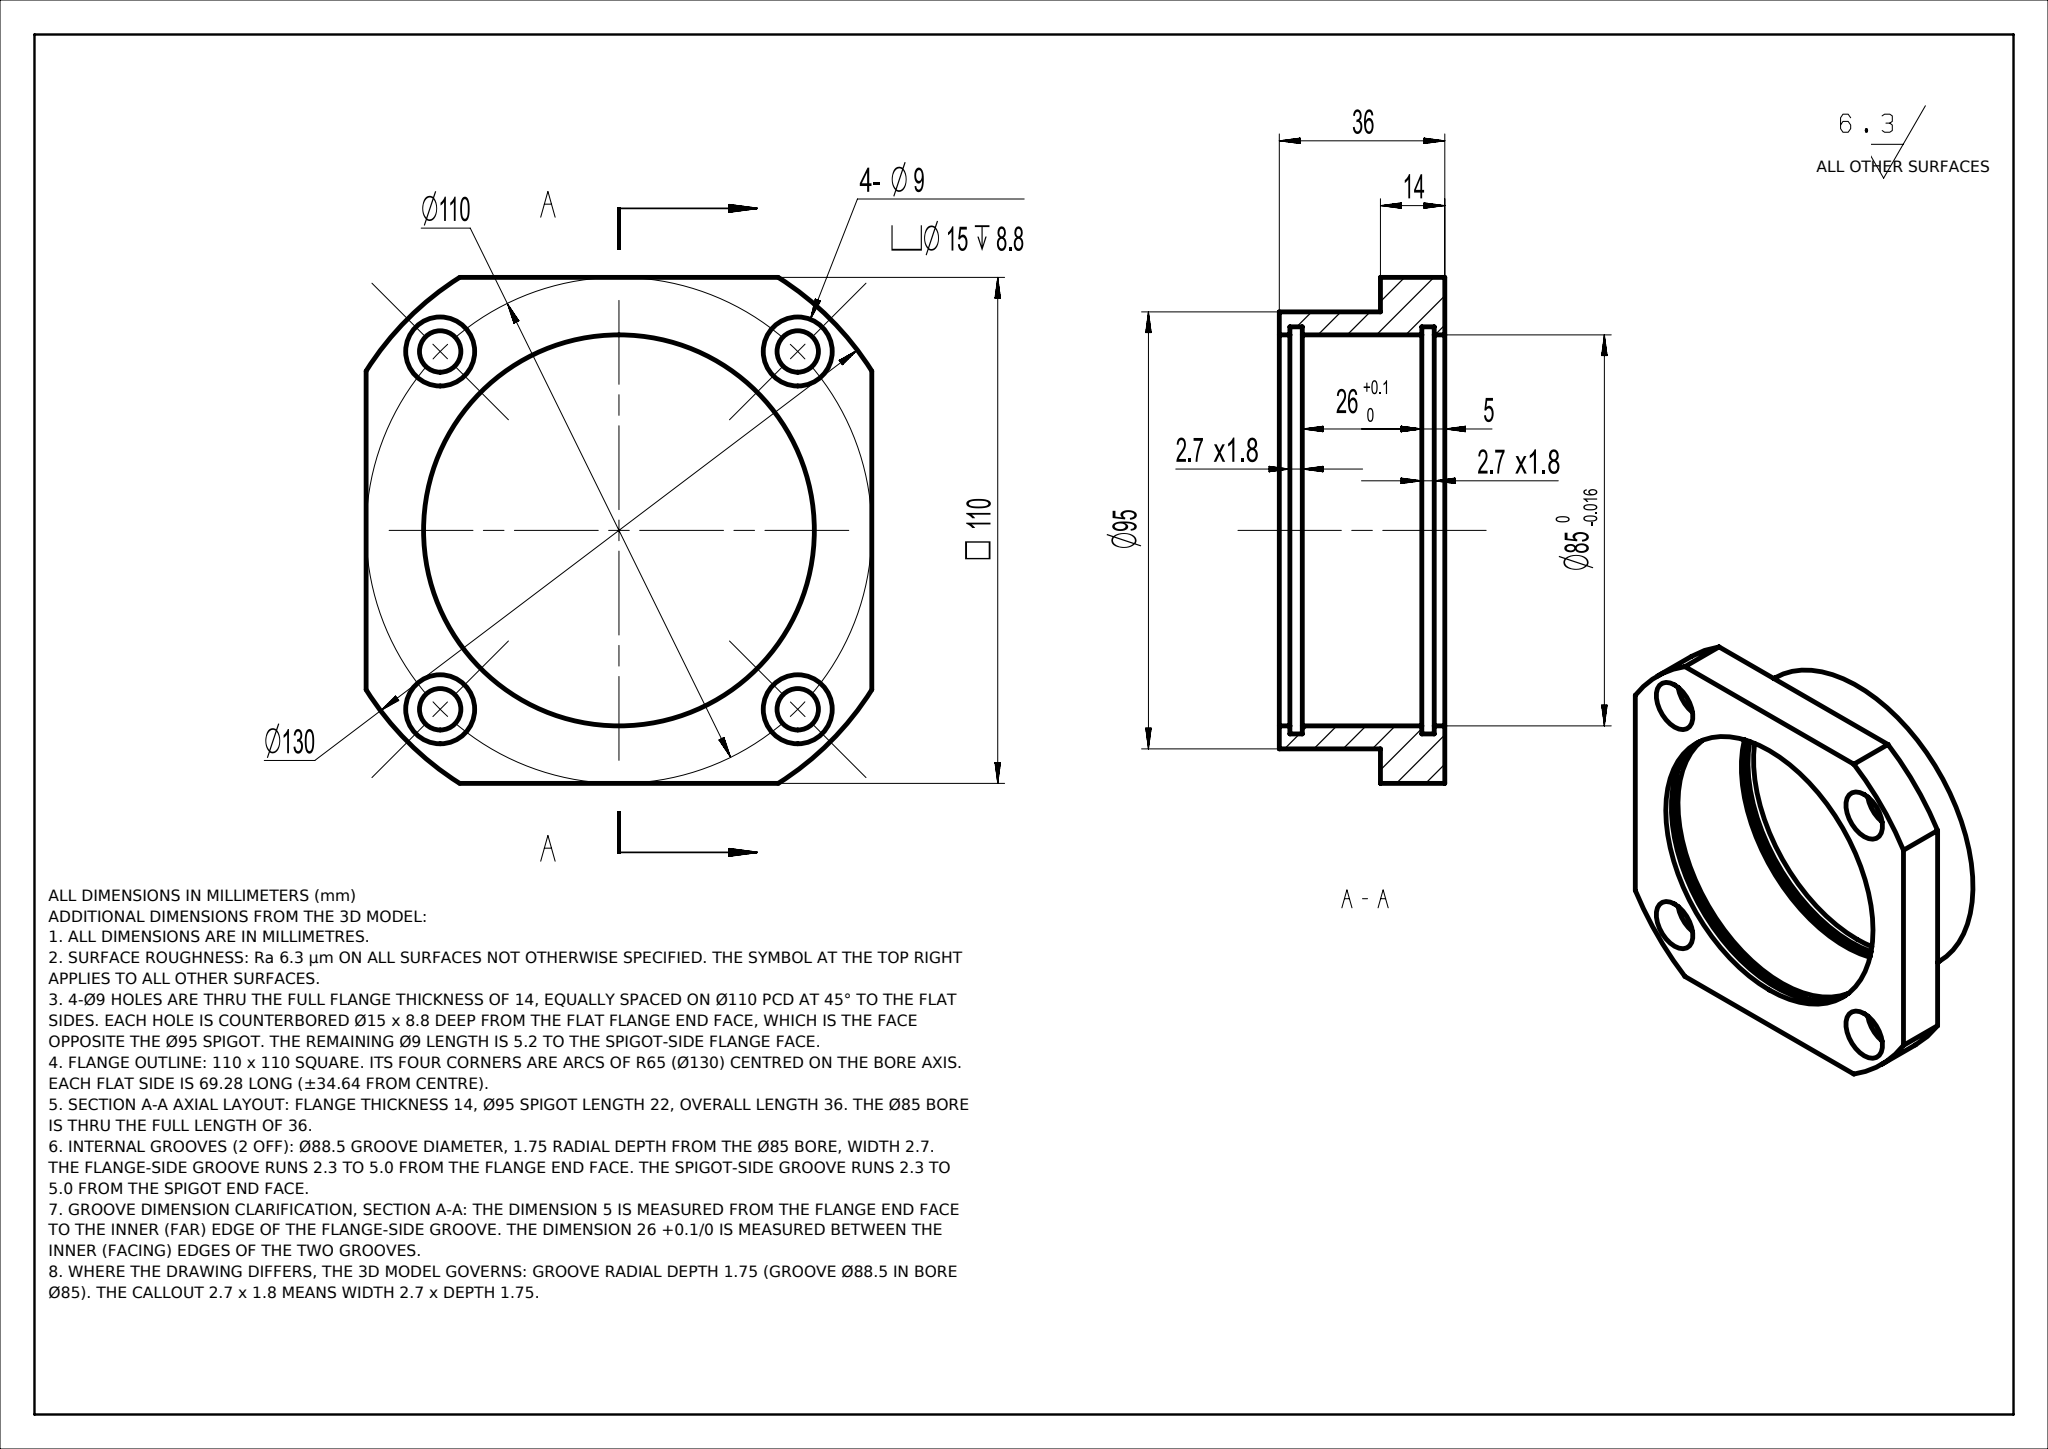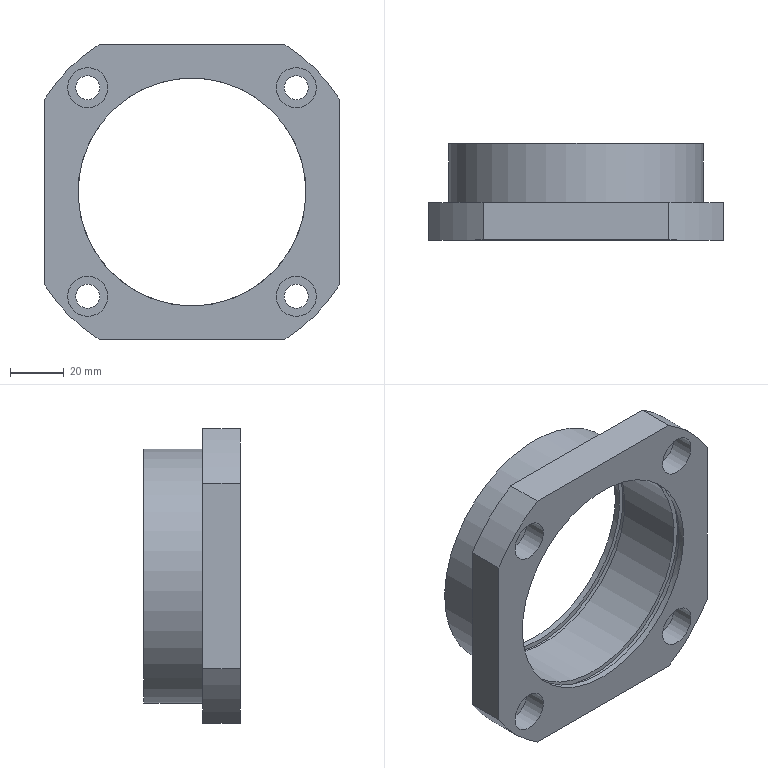Part | NX | mm | 1 solid | 33 faces | box 110 x 36 x 110 mm | volume 101074 mm3 | cylinder 18 | plane 15 | commonest cylinder face diameters 130 x4 9 x4 15 x4 85 x3 88.5 x2 95 x1
STEP:
#1=CARTESIAN_POINT('',(0.,0.,0.));
#2=DIRECTION('',(0.,0.,1.));
#3=DIRECTION('',(1.,0.,0.));
#4=AXIS2_PLACEMENT_3D('',#1,#2,#3);
#5=(LENGTH_UNIT()NAMED_UNIT(*)SI_UNIT(.MILLI.,.METRE.));
#6=UNCERTAINTY_MEASURE_WITH_UNIT(LENGTH_MEASURE(0.00002),#5,'','');
#7=(NAMED_UNIT(*)PLANE_ANGLE_UNIT()SI_UNIT($,.RADIAN.));
#8=PLANE_ANGLE_MEASURE_WITH_UNIT(PLANE_ANGLE_MEASURE(0.01745),#7);
#9=DIMENSIONAL_EXPONENTS(0.,0.,0.,0.,0.,0.,0.);
#10=(CONVERSION_BASED_UNIT('',#8)NAMED_UNIT(#9)PLANE_ANGLE_UNIT());
#11=(NAMED_UNIT(*)SI_UNIT($,.STERADIAN.)SOLID_ANGLE_UNIT());
#12=(GEOMETRIC_REPRESENTATION_CONTEXT(3)GLOBAL_UNCERTAINTY_ASSIGNED_CONTEXT((#6))GLOBAL_UNIT_ASSIGNED_CONTEXT((#5,#10,#11))REPRESENTATION_CONTEXT('',''));
#13=SHAPE_REPRESENTATION('',(#4),#12);
#14=CARTESIAN_POINT('',(-34.641,12.426,55.));
#15=VERTEX_POINT('',#14);
#16=CARTESIAN_POINT('',(-55.,12.426,34.641));
#17=VERTEX_POINT('',#16);
#18=CARTESIAN_POINT('',(0.,12.426,0.));
#19=DIRECTION('',(0.,-1.,0.));
#20=DIRECTION('',(0.,0.,-1.));
#21=AXIS2_PLACEMENT_3D('',#18,#19,#20);
#22=CIRCLE('',#21,65.);
#23=EDGE_CURVE('',#15,#17,#22,.T.);
#24=ORIENTED_EDGE('',*,*,#23,.T.);
#25=CARTESIAN_POINT('',(-55.,-1.574,34.641));
#26=VERTEX_POINT('',#25);
#27=CARTESIAN_POINT('',(-55.,0.,34.641));
#28=DIRECTION('',(0.,-1.,0.));
#29=VECTOR('',#28,1.);
#30=LINE('',#27,#29);
#31=EDGE_CURVE('',#17,#26,#30,.T.);
#32=ORIENTED_EDGE('',*,*,#31,.T.);
#33=CARTESIAN_POINT('',(-34.641,-1.574,55.));
#34=VERTEX_POINT('',#33);
#35=CARTESIAN_POINT('',(0.,-1.574,0.));
#36=DIRECTION('',(0.,-1.,0.));
#37=DIRECTION('',(0.,0.,-1.));
#38=AXIS2_PLACEMENT_3D('',#35,#36,#37);
#39=CIRCLE('',#38,65.);
#40=EDGE_CURVE('',#34,#26,#39,.T.);
#41=ORIENTED_EDGE('',*,*,#40,.F.);
#42=CARTESIAN_POINT('',(-34.641,0.,55.));
#43=DIRECTION('',(0.,1.,0.));
#44=VECTOR('',#43,1.);
#45=LINE('',#42,#44);
#46=EDGE_CURVE('',#34,#15,#45,.T.);
#47=ORIENTED_EDGE('',*,*,#46,.T.);
#48=EDGE_LOOP('',(#24,#32,#41,#47));
#49=FACE_OUTER_BOUND('',#48,.T.);
#50=CARTESIAN_POINT('',(0.,0.,0.));
#51=DIRECTION('',(0.,-1.,0.));
#52=DIRECTION('',(0.,0.,-1.));
#53=AXIS2_PLACEMENT_3D('',#50,#51,#52);
#54=CYLINDRICAL_SURFACE('',#53,65.);
#55=ADVANCED_FACE('',(#49),#54,.T.);
#56=CARTESIAN_POINT('',(-55.,-1.574,-34.641));
#57=VERTEX_POINT('',#56);
#58=CARTESIAN_POINT('',(-34.641,-1.574,-55.));
#59=VERTEX_POINT('',#58);
#60=CARTESIAN_POINT('',(0.,-1.574,0.));
#61=DIRECTION('',(0.,-1.,0.));
#62=DIRECTION('',(0.,0.,-1.));
#63=AXIS2_PLACEMENT_3D('',#60,#61,#62);
#64=CIRCLE('',#63,65.);
#65=EDGE_CURVE('',#57,#59,#64,.T.);
#66=ORIENTED_EDGE('',*,*,#65,.F.);
#67=CARTESIAN_POINT('',(-55.,12.426,-34.641));
#68=VERTEX_POINT('',#67);
#69=CARTESIAN_POINT('',(-55.,0.,-34.641));
#70=DIRECTION('',(0.,1.,0.));
#71=VECTOR('',#70,1.);
#72=LINE('',#69,#71);
#73=EDGE_CURVE('',#57,#68,#72,.T.);
#74=ORIENTED_EDGE('',*,*,#73,.T.);
#75=CARTESIAN_POINT('',(-34.641,12.426,-55.));
#76=VERTEX_POINT('',#75);
#77=CARTESIAN_POINT('',(0.,12.426,0.));
#78=DIRECTION('',(0.,-1.,0.));
#79=DIRECTION('',(0.,0.,-1.));
#80=AXIS2_PLACEMENT_3D('',#77,#78,#79);
#81=CIRCLE('',#80,65.);
#82=EDGE_CURVE('',#68,#76,#81,.T.);
#83=ORIENTED_EDGE('',*,*,#82,.T.);
#84=CARTESIAN_POINT('',(-34.641,0.,-55.));
#85=DIRECTION('',(0.,-1.,0.));
#86=VECTOR('',#85,1.);
#87=LINE('',#84,#86);
#88=EDGE_CURVE('',#76,#59,#87,.T.);
#89=ORIENTED_EDGE('',*,*,#88,.T.);
#90=EDGE_LOOP('',(#66,#74,#83,#89));
#91=FACE_OUTER_BOUND('',#90,.T.);
#92=CARTESIAN_POINT('',(0.,0.,0.));
#93=DIRECTION('',(0.,-1.,0.));
#94=DIRECTION('',(0.,0.,-1.));
#95=AXIS2_PLACEMENT_3D('',#92,#93,#94);
#96=CYLINDRICAL_SURFACE('',#95,65.);
#97=ADVANCED_FACE('',(#91),#96,.T.);
#98=CARTESIAN_POINT('',(34.641,-1.574,-55.));
#99=VERTEX_POINT('',#98);
#100=CARTESIAN_POINT('',(55.,-1.574,-34.641));
#101=VERTEX_POINT('',#100);
#102=CARTESIAN_POINT('',(0.,-1.574,0.));
#103=DIRECTION('',(0.,-1.,0.));
#104=DIRECTION('',(0.,0.,-1.));
#105=AXIS2_PLACEMENT_3D('',#102,#103,#104);
#106=CIRCLE('',#105,65.);
#107=EDGE_CURVE('',#99,#101,#106,.T.);
#108=ORIENTED_EDGE('',*,*,#107,.F.);
#109=CARTESIAN_POINT('',(34.641,12.426,-55.));
#110=VERTEX_POINT('',#109);
#111=CARTESIAN_POINT('',(34.641,0.,-55.));
#112=DIRECTION('',(0.,1.,0.));
#113=VECTOR('',#112,1.);
#114=LINE('',#111,#113);
#115=EDGE_CURVE('',#99,#110,#114,.T.);
#116=ORIENTED_EDGE('',*,*,#115,.T.);
#117=CARTESIAN_POINT('',(55.,12.426,-34.641));
#118=VERTEX_POINT('',#117);
#119=CARTESIAN_POINT('',(0.,12.426,0.));
#120=DIRECTION('',(0.,-1.,0.));
#121=DIRECTION('',(0.,0.,-1.));
#122=AXIS2_PLACEMENT_3D('',#119,#120,#121);
#123=CIRCLE('',#122,65.);
#124=EDGE_CURVE('',#110,#118,#123,.T.);
#125=ORIENTED_EDGE('',*,*,#124,.T.);
#126=CARTESIAN_POINT('',(55.,0.,-34.641));
#127=DIRECTION('',(0.,-1.,0.));
#128=VECTOR('',#127,1.);
#129=LINE('',#126,#128);
#130=EDGE_CURVE('',#118,#101,#129,.T.);
#131=ORIENTED_EDGE('',*,*,#130,.T.);
#132=EDGE_LOOP('',(#108,#116,#125,#131));
#133=FACE_OUTER_BOUND('',#132,.T.);
#134=CARTESIAN_POINT('',(0.,0.,0.));
#135=DIRECTION('',(0.,-1.,0.));
#136=DIRECTION('',(0.,0.,-1.));
#137=AXIS2_PLACEMENT_3D('',#134,#135,#136);
#138=CYLINDRICAL_SURFACE('',#137,65.);
#139=ADVANCED_FACE('',(#133),#138,.T.);
#140=CARTESIAN_POINT('',(0.,3.426,42.5));
#141=VERTEX_POINT('',#140);
#142=CARTESIAN_POINT('',(0.,3.426,0.));
#143=DIRECTION('',(0.,-1.,0.));
#144=DIRECTION('',(0.,0.,1.));
#145=AXIS2_PLACEMENT_3D('',#142,#143,#144);
#146=CIRCLE('',#145,42.5);
#147=EDGE_CURVE('',#141,#141,#146,.T.);
#148=ORIENTED_EDGE('',*,*,#147,.T.);
#149=EDGE_LOOP('',(#148));
#150=FACE_BOUND('',#149,.T.);
#151=CARTESIAN_POINT('',(0.,29.426,42.5));
#152=VERTEX_POINT('',#151);
#153=CARTESIAN_POINT('',(0.,29.426,0.));
#154=DIRECTION('',(0.,-1.,0.));
#155=DIRECTION('',(0.,0.,1.));
#156=AXIS2_PLACEMENT_3D('',#153,#154,#155);
#157=CIRCLE('',#156,42.5);
#158=EDGE_CURVE('',#152,#152,#157,.T.);
#159=ORIENTED_EDGE('',*,*,#158,.F.);
#160=EDGE_LOOP('',(#159));
#161=FACE_BOUND('',#160,.T.);
#162=CARTESIAN_POINT('',(0.,0.,0.));
#163=DIRECTION('',(0.,-1.,0.));
#164=DIRECTION('',(0.,0.,-1.));
#165=AXIS2_PLACEMENT_3D('',#162,#163,#164);
#166=CYLINDRICAL_SURFACE('',#165,42.5);
#167=ADVANCED_FACE('',(#150,#161),#166,.F.);
#168=CARTESIAN_POINT('',(0.,-1.574,-42.5));
#169=VERTEX_POINT('',#168);
#170=CARTESIAN_POINT('',(0.,-1.574,0.));
#171=DIRECTION('',(0.,-1.,0.));
#172=DIRECTION('',(0.,0.,-1.));
#173=AXIS2_PLACEMENT_3D('',#170,#171,#172);
#174=CIRCLE('',#173,42.5);
#175=EDGE_CURVE('',#169,#169,#174,.T.);
#176=ORIENTED_EDGE('',*,*,#175,.T.);
#177=EDGE_LOOP('',(#176));
#178=FACE_BOUND('',#177,.T.);
#179=CARTESIAN_POINT('',(0.,0.7259,42.5));
#180=VERTEX_POINT('',#179);
#181=CARTESIAN_POINT('',(0.,0.7259,0.));
#182=DIRECTION('',(0.,-1.,0.));
#183=DIRECTION('',(0.,0.,1.));
#184=AXIS2_PLACEMENT_3D('',#181,#182,#183);
#185=CIRCLE('',#184,42.5);
#186=EDGE_CURVE('',#180,#180,#185,.T.);
#187=ORIENTED_EDGE('',*,*,#186,.F.);
#188=EDGE_LOOP('',(#187));
#189=FACE_BOUND('',#188,.T.);
#190=CARTESIAN_POINT('',(0.,0.,0.));
#191=DIRECTION('',(0.,-1.,0.));
#192=DIRECTION('',(0.,0.,-1.));
#193=AXIS2_PLACEMENT_3D('',#190,#191,#192);
#194=CYLINDRICAL_SURFACE('',#193,42.5);
#195=ADVANCED_FACE('',(#178,#189),#194,.F.);
#196=CARTESIAN_POINT('',(38.891,-1.574,46.391));
#197=VERTEX_POINT('',#196);
#198=CARTESIAN_POINT('',(38.891,-1.574,38.891));
#199=DIRECTION('',(0.,1.,0.));
#200=DIRECTION('',(0.,0.,1.));
#201=AXIS2_PLACEMENT_3D('',#198,#199,#200);
#202=CIRCLE('',#201,7.5);
#203=EDGE_CURVE('',#197,#197,#202,.T.);
#204=ORIENTED_EDGE('',*,*,#203,.T.);
#205=EDGE_LOOP('',(#204));
#206=FACE_BOUND('',#205,.T.);
#207=CARTESIAN_POINT('',(38.891,-1.574,-31.391));
#208=VERTEX_POINT('',#207);
#209=CARTESIAN_POINT('',(38.891,-1.574,-38.891));
#210=DIRECTION('',(0.,1.,0.));
#211=DIRECTION('',(0.,0.,1.));
#212=AXIS2_PLACEMENT_3D('',#209,#210,#211);
#213=CIRCLE('',#212,7.5);
#214=EDGE_CURVE('',#208,#208,#213,.T.);
#215=ORIENTED_EDGE('',*,*,#214,.T.);
#216=EDGE_LOOP('',(#215));
#217=FACE_BOUND('',#216,.T.);
#218=CARTESIAN_POINT('',(-38.891,-1.574,46.391));
#219=VERTEX_POINT('',#218);
#220=CARTESIAN_POINT('',(-38.891,-1.574,38.891));
#221=DIRECTION('',(0.,1.,0.));
#222=DIRECTION('',(0.,0.,1.));
#223=AXIS2_PLACEMENT_3D('',#220,#221,#222);
#224=CIRCLE('',#223,7.5);
#225=EDGE_CURVE('',#219,#219,#224,.T.);
#226=ORIENTED_EDGE('',*,*,#225,.T.);
#227=EDGE_LOOP('',(#226));
#228=FACE_BOUND('',#227,.T.);
#229=CARTESIAN_POINT('',(-38.891,-1.574,-31.391));
#230=VERTEX_POINT('',#229);
#231=CARTESIAN_POINT('',(-38.891,-1.574,-38.891));
#232=DIRECTION('',(0.,1.,0.));
#233=DIRECTION('',(0.,0.,1.));
#234=AXIS2_PLACEMENT_3D('',#231,#232,#233);
#235=CIRCLE('',#234,7.5);
#236=EDGE_CURVE('',#230,#230,#235,.T.);
#237=ORIENTED_EDGE('',*,*,#236,.T.);
#238=EDGE_LOOP('',(#237));
#239=FACE_BOUND('',#238,.T.);
#240=ORIENTED_EDGE('',*,*,#175,.F.);
#241=EDGE_LOOP('',(#240));
#242=FACE_BOUND('',#241,.T.);
#243=CARTESIAN_POINT('',(55.,-1.574,34.641));
#244=VERTEX_POINT('',#243);
#245=CARTESIAN_POINT('',(34.641,-1.574,55.));
#246=VERTEX_POINT('',#245);
#247=CARTESIAN_POINT('',(0.,-1.574,0.));
#248=DIRECTION('',(0.,-1.,0.));
#249=DIRECTION('',(0.,0.,-1.));
#250=AXIS2_PLACEMENT_3D('',#247,#248,#249);
#251=CIRCLE('',#250,65.);
#252=EDGE_CURVE('',#244,#246,#251,.T.);
#253=ORIENTED_EDGE('',*,*,#252,.T.);
#254=CARTESIAN_POINT('',(55.,-1.574,55.));
#255=DIRECTION('',(-1.,0.,0.));
#256=VECTOR('',#255,1.);
#257=LINE('',#254,#256);
#258=EDGE_CURVE('',#246,#34,#257,.T.);
#259=ORIENTED_EDGE('',*,*,#258,.T.);
#260=ORIENTED_EDGE('',*,*,#40,.T.);
#261=CARTESIAN_POINT('',(-55.,-1.574,55.));
#262=DIRECTION('',(-0.,0.,-1.));
#263=VECTOR('',#262,1.);
#264=LINE('',#261,#263);
#265=EDGE_CURVE('',#26,#57,#264,.T.);
#266=ORIENTED_EDGE('',*,*,#265,.T.);
#267=ORIENTED_EDGE('',*,*,#65,.T.);
#268=CARTESIAN_POINT('',(-55.,-1.574,-55.));
#269=DIRECTION('',(1.,0.,-0.));
#270=VECTOR('',#269,1.);
#271=LINE('',#268,#270);
#272=EDGE_CURVE('',#59,#99,#271,.T.);
#273=ORIENTED_EDGE('',*,*,#272,.T.);
#274=ORIENTED_EDGE('',*,*,#107,.T.);
#275=CARTESIAN_POINT('',(55.,-1.574,-55.));
#276=DIRECTION('',(0.,0.,1.));
#277=VECTOR('',#276,1.);
#278=LINE('',#275,#277);
#279=EDGE_CURVE('',#101,#244,#278,.T.);
#280=ORIENTED_EDGE('',*,*,#279,.T.);
#281=EDGE_LOOP('',(#253,#259,#260,#266,#267,#273,#274,#280));
#282=FACE_BOUND('',#281,.T.);
#283=CARTESIAN_POINT('',(0.,-1.574,65.));
#284=DIRECTION('',(0.,1.,0.));
#285=DIRECTION('',(0.,0.,1.));
#286=AXIS2_PLACEMENT_3D('',#283,#284,#285);
#287=PLANE('',#286);
#288=ADVANCED_FACE('',(#206,#217,#228,#239,#242,#282),#287,.F.);
#289=CARTESIAN_POINT('',(0.,32.126,42.5));
#290=VERTEX_POINT('',#289);
#291=CARTESIAN_POINT('',(0.,32.126,0.));
#292=DIRECTION('',(0.,-1.,0.));
#293=DIRECTION('',(0.,0.,1.));
#294=AXIS2_PLACEMENT_3D('',#291,#292,#293);
#295=CIRCLE('',#294,42.5);
#296=EDGE_CURVE('',#290,#290,#295,.T.);
#297=ORIENTED_EDGE('',*,*,#296,.T.);
#298=EDGE_LOOP('',(#297));
#299=FACE_BOUND('',#298,.T.);
#300=CARTESIAN_POINT('',(0.,34.426,-42.5));
#301=VERTEX_POINT('',#300);
#302=CARTESIAN_POINT('',(0.,34.426,0.));
#303=DIRECTION('',(0.,-1.,0.));
#304=DIRECTION('',(0.,0.,-1.));
#305=AXIS2_PLACEMENT_3D('',#302,#303,#304);
#306=CIRCLE('',#305,42.5);
#307=EDGE_CURVE('',#301,#301,#306,.T.);
#308=ORIENTED_EDGE('',*,*,#307,.F.);
#309=EDGE_LOOP('',(#308));
#310=FACE_BOUND('',#309,.T.);
#311=CARTESIAN_POINT('',(0.,0.,0.));
#312=DIRECTION('',(0.,-1.,0.));
#313=DIRECTION('',(0.,0.,-1.));
#314=AXIS2_PLACEMENT_3D('',#311,#312,#313);
#315=CYLINDRICAL_SURFACE('',#314,42.5);
#316=ADVANCED_FACE('',(#299,#310),#315,.F.);
#317=CARTESIAN_POINT('',(0.,34.426,-47.5));
#318=VERTEX_POINT('',#317);
#319=CARTESIAN_POINT('',(0.,34.426,0.));
#320=DIRECTION('',(0.,-1.,0.));
#321=DIRECTION('',(0.,0.,-1.));
#322=AXIS2_PLACEMENT_3D('',#319,#320,#321);
#323=CIRCLE('',#322,47.5);
#324=EDGE_CURVE('',#318,#318,#323,.T.);
#325=ORIENTED_EDGE('',*,*,#324,.F.);
#326=EDGE_LOOP('',(#325));
#327=FACE_BOUND('',#326,.T.);
#328=ORIENTED_EDGE('',*,*,#307,.T.);
#329=EDGE_LOOP('',(#328));
#330=FACE_BOUND('',#329,.T.);
#331=CARTESIAN_POINT('',(0.,34.426,42.5));
#332=DIRECTION('',(0.,-1.,0.));
#333=DIRECTION('',(0.,0.,-1.));
#334=AXIS2_PLACEMENT_3D('',#331,#332,#333);
#335=PLANE('',#334);
#336=ADVANCED_FACE('',(#327,#330),#335,.F.);
#337=CARTESIAN_POINT('',(0.,12.426,-47.5));
#338=VERTEX_POINT('',#337);
#339=CARTESIAN_POINT('',(0.,12.426,0.));
#340=DIRECTION('',(0.,-1.,0.));
#341=DIRECTION('',(0.,0.,-1.));
#342=AXIS2_PLACEMENT_3D('',#339,#340,#341);
#343=CIRCLE('',#342,47.5);
#344=EDGE_CURVE('',#338,#338,#343,.T.);
#345=ORIENTED_EDGE('',*,*,#344,.F.);
#346=EDGE_LOOP('',(#345));
#347=FACE_BOUND('',#346,.T.);
#348=ORIENTED_EDGE('',*,*,#324,.T.);
#349=EDGE_LOOP('',(#348));
#350=FACE_BOUND('',#349,.T.);
#351=CARTESIAN_POINT('',(0.,0.,0.));
#352=DIRECTION('',(0.,-1.,0.));
#353=DIRECTION('',(0.,0.,-1.));
#354=AXIS2_PLACEMENT_3D('',#351,#352,#353);
#355=CYLINDRICAL_SURFACE('',#354,47.5);
#356=ADVANCED_FACE('',(#347,#350),#355,.T.);
#357=CARTESIAN_POINT('',(38.891,12.426,34.391));
#358=VERTEX_POINT('',#357);
#359=CARTESIAN_POINT('',(38.891,12.426,38.891));
#360=DIRECTION('',(0.,-1.,0.));
#361=DIRECTION('',(0.,0.,-1.));
#362=AXIS2_PLACEMENT_3D('',#359,#360,#361);
#363=CIRCLE('',#362,4.5);
#364=EDGE_CURVE('',#358,#358,#363,.T.);
#365=ORIENTED_EDGE('',*,*,#364,.T.);
#366=EDGE_LOOP('',(#365));
#367=FACE_BOUND('',#366,.T.);
#368=CARTESIAN_POINT('',(38.891,12.426,-43.391));
#369=VERTEX_POINT('',#368);
#370=CARTESIAN_POINT('',(38.891,12.426,-38.891));
#371=DIRECTION('',(0.,-1.,0.));
#372=DIRECTION('',(0.,0.,-1.));
#373=AXIS2_PLACEMENT_3D('',#370,#371,#372);
#374=CIRCLE('',#373,4.5);
#375=EDGE_CURVE('',#369,#369,#374,.T.);
#376=ORIENTED_EDGE('',*,*,#375,.T.);
#377=EDGE_LOOP('',(#376));
#378=FACE_BOUND('',#377,.T.);
#379=CARTESIAN_POINT('',(-38.891,12.426,34.391));
#380=VERTEX_POINT('',#379);
#381=CARTESIAN_POINT('',(-38.891,12.426,38.891));
#382=DIRECTION('',(0.,-1.,0.));
#383=DIRECTION('',(0.,0.,-1.));
#384=AXIS2_PLACEMENT_3D('',#381,#382,#383);
#385=CIRCLE('',#384,4.5);
#386=EDGE_CURVE('',#380,#380,#385,.T.);
#387=ORIENTED_EDGE('',*,*,#386,.T.);
#388=EDGE_LOOP('',(#387));
#389=FACE_BOUND('',#388,.T.);
#390=CARTESIAN_POINT('',(-38.891,12.426,-43.391));
#391=VERTEX_POINT('',#390);
#392=CARTESIAN_POINT('',(-38.891,12.426,-38.891));
#393=DIRECTION('',(0.,-1.,0.));
#394=DIRECTION('',(0.,0.,-1.));
#395=AXIS2_PLACEMENT_3D('',#392,#393,#394);
#396=CIRCLE('',#395,4.5);
#397=EDGE_CURVE('',#391,#391,#396,.T.);
#398=ORIENTED_EDGE('',*,*,#397,.T.);
#399=EDGE_LOOP('',(#398));
#400=FACE_BOUND('',#399,.T.);
#401=ORIENTED_EDGE('',*,*,#82,.F.);
#402=CARTESIAN_POINT('',(-55.,12.426,47.5));
#403=DIRECTION('',(0.,0.,1.));
#404=VECTOR('',#403,1.);
#405=LINE('',#402,#404);
#406=EDGE_CURVE('',#68,#17,#405,.T.);
#407=ORIENTED_EDGE('',*,*,#406,.T.);
#408=ORIENTED_EDGE('',*,*,#23,.F.);
#409=CARTESIAN_POINT('',(34.641,12.426,55.));
#410=VERTEX_POINT('',#409);
#411=CARTESIAN_POINT('',(0.,12.426,55.));
#412=DIRECTION('',(1.,0.,-0.));
#413=VECTOR('',#412,1.);
#414=LINE('',#411,#413);
#415=EDGE_CURVE('',#15,#410,#414,.T.);
#416=ORIENTED_EDGE('',*,*,#415,.T.);
#417=CARTESIAN_POINT('',(55.,12.426,34.641));
#418=VERTEX_POINT('',#417);
#419=CARTESIAN_POINT('',(0.,12.426,0.));
#420=DIRECTION('',(0.,-1.,0.));
#421=DIRECTION('',(0.,0.,-1.));
#422=AXIS2_PLACEMENT_3D('',#419,#420,#421);
#423=CIRCLE('',#422,65.);
#424=EDGE_CURVE('',#418,#410,#423,.T.);
#425=ORIENTED_EDGE('',*,*,#424,.F.);
#426=CARTESIAN_POINT('',(55.,12.426,47.5));
#427=DIRECTION('',(-0.,0.,-1.));
#428=VECTOR('',#427,1.);
#429=LINE('',#426,#428);
#430=EDGE_CURVE('',#418,#118,#429,.T.);
#431=ORIENTED_EDGE('',*,*,#430,.T.);
#432=ORIENTED_EDGE('',*,*,#124,.F.);
#433=CARTESIAN_POINT('',(-0.,12.426,-55.));
#434=DIRECTION('',(-1.,0.,0.));
#435=VECTOR('',#434,1.);
#436=LINE('',#433,#435);
#437=EDGE_CURVE('',#110,#76,#436,.T.);
#438=ORIENTED_EDGE('',*,*,#437,.T.);
#439=EDGE_LOOP('',(#401,#407,#408,#416,#425,#431,#432,#438));
#440=FACE_BOUND('',#439,.T.);
#441=ORIENTED_EDGE('',*,*,#344,.T.);
#442=EDGE_LOOP('',(#441));
#443=FACE_BOUND('',#442,.T.);
#444=CARTESIAN_POINT('',(0.,12.426,47.5));
#445=DIRECTION('',(0.,-1.,0.));
#446=DIRECTION('',(0.,0.,-1.));
#447=AXIS2_PLACEMENT_3D('',#444,#445,#446);
#448=PLANE('',#447);
#449=ADVANCED_FACE('',(#367,#378,#389,#400,#440,#443),#448,.F.);
#450=ORIENTED_EDGE('',*,*,#252,.F.);
#451=CARTESIAN_POINT('',(55.,0.,34.641));
#452=DIRECTION('',(0.,1.,0.));
#453=VECTOR('',#452,1.);
#454=LINE('',#451,#453);
#455=EDGE_CURVE('',#244,#418,#454,.T.);
#456=ORIENTED_EDGE('',*,*,#455,.T.);
#457=ORIENTED_EDGE('',*,*,#424,.T.);
#458=CARTESIAN_POINT('',(34.641,0.,55.));
#459=DIRECTION('',(0.,-1.,0.));
#460=VECTOR('',#459,1.);
#461=LINE('',#458,#460);
#462=EDGE_CURVE('',#410,#246,#461,.T.);
#463=ORIENTED_EDGE('',*,*,#462,.T.);
#464=EDGE_LOOP('',(#450,#456,#457,#463));
#465=FACE_OUTER_BOUND('',#464,.T.);
#466=CARTESIAN_POINT('',(0.,0.,0.));
#467=DIRECTION('',(0.,-1.,0.));
#468=DIRECTION('',(0.,0.,-1.));
#469=AXIS2_PLACEMENT_3D('',#466,#467,#468);
#470=CYLINDRICAL_SURFACE('',#469,65.);
#471=ADVANCED_FACE('',(#465),#470,.T.);
#472=CARTESIAN_POINT('',(0.,0.7259,44.25));
#473=VERTEX_POINT('',#472);
#474=CARTESIAN_POINT('',(0.,0.7259,0.));
#475=DIRECTION('',(0.,-1.,0.));
#476=DIRECTION('',(0.,0.,1.));
#477=AXIS2_PLACEMENT_3D('',#474,#475,#476);
#478=CIRCLE('',#477,44.25);
#479=EDGE_CURVE('',#473,#473,#478,.T.);
#480=ORIENTED_EDGE('',*,*,#479,.F.);
#481=EDGE_LOOP('',(#480));
#482=FACE_BOUND('',#481,.T.);
#483=ORIENTED_EDGE('',*,*,#186,.T.);
#484=EDGE_LOOP('',(#483));
#485=FACE_BOUND('',#484,.T.);
#486=CARTESIAN_POINT('',(0.,0.7259,0.));
#487=DIRECTION('',(0.,1.,0.));
#488=DIRECTION('',(0.,0.,1.));
#489=AXIS2_PLACEMENT_3D('',#486,#487,#488);
#490=PLANE('',#489);
#491=ADVANCED_FACE('',(#482,#485),#490,.T.);
#492=CARTESIAN_POINT('',(0.,3.426,44.25));
#493=VERTEX_POINT('',#492);
#494=CARTESIAN_POINT('',(0.,3.426,0.));
#495=DIRECTION('',(0.,-1.,0.));
#496=DIRECTION('',(0.,0.,1.));
#497=AXIS2_PLACEMENT_3D('',#494,#495,#496);
#498=CIRCLE('',#497,44.25);
#499=EDGE_CURVE('',#493,#493,#498,.T.);
#500=ORIENTED_EDGE('',*,*,#499,.T.);
#501=EDGE_LOOP('',(#500));
#502=FACE_BOUND('',#501,.T.);
#503=ORIENTED_EDGE('',*,*,#147,.F.);
#504=EDGE_LOOP('',(#503));
#505=FACE_BOUND('',#504,.T.);
#506=CARTESIAN_POINT('',(0.,3.426,0.));
#507=DIRECTION('',(0.,1.,0.));
#508=DIRECTION('',(0.,0.,1.));
#509=AXIS2_PLACEMENT_3D('',#506,#507,#508);
#510=PLANE('',#509);
#511=ADVANCED_FACE('',(#502,#505),#510,.F.);
#512=ORIENTED_EDGE('',*,*,#499,.F.);
#513=EDGE_LOOP('',(#512));
#514=FACE_BOUND('',#513,.T.);
#515=ORIENTED_EDGE('',*,*,#479,.T.);
#516=EDGE_LOOP('',(#515));
#517=FACE_BOUND('',#516,.T.);
#518=CARTESIAN_POINT('',(0.,2.076,0.));
#519=DIRECTION('',(0.,1.,0.));
#520=DIRECTION('',(0.,0.,1.));
#521=AXIS2_PLACEMENT_3D('',#518,#519,#520);
#522=CYLINDRICAL_SURFACE('',#521,44.25);
#523=ADVANCED_FACE('',(#514,#517),#522,.F.);
#524=CARTESIAN_POINT('',(0.,32.126,44.25));
#525=VERTEX_POINT('',#524);
#526=CARTESIAN_POINT('',(0.,32.126,0.));
#527=DIRECTION('',(0.,-1.,0.));
#528=DIRECTION('',(0.,0.,1.));
#529=AXIS2_PLACEMENT_3D('',#526,#527,#528);
#530=CIRCLE('',#529,44.25);
#531=EDGE_CURVE('',#525,#525,#530,.T.);
#532=ORIENTED_EDGE('',*,*,#531,.T.);
#533=EDGE_LOOP('',(#532));
#534=FACE_BOUND('',#533,.T.);
#535=ORIENTED_EDGE('',*,*,#296,.F.);
#536=EDGE_LOOP('',(#535));
#537=FACE_BOUND('',#536,.T.);
#538=CARTESIAN_POINT('',(0.,32.126,0.));
#539=DIRECTION('',(0.,1.,0.));
#540=DIRECTION('',(0.,0.,1.));
#541=AXIS2_PLACEMENT_3D('',#538,#539,#540);
#542=PLANE('',#541);
#543=ADVANCED_FACE('',(#534,#537),#542,.F.);
#544=CARTESIAN_POINT('',(0.,29.426,44.25));
#545=VERTEX_POINT('',#544);
#546=CARTESIAN_POINT('',(0.,29.426,0.));
#547=DIRECTION('',(0.,-1.,0.));
#548=DIRECTION('',(0.,0.,1.));
#549=AXIS2_PLACEMENT_3D('',#546,#547,#548);
#550=CIRCLE('',#549,44.25);
#551=EDGE_CURVE('',#545,#545,#550,.T.);
#552=ORIENTED_EDGE('',*,*,#551,.F.);
#553=EDGE_LOOP('',(#552));
#554=FACE_BOUND('',#553,.T.);
#555=ORIENTED_EDGE('',*,*,#158,.T.);
#556=EDGE_LOOP('',(#555));
#557=FACE_BOUND('',#556,.T.);
#558=CARTESIAN_POINT('',(0.,29.426,0.));
#559=DIRECTION('',(0.,1.,0.));
#560=DIRECTION('',(0.,0.,1.));
#561=AXIS2_PLACEMENT_3D('',#558,#559,#560);
#562=PLANE('',#561);
#563=ADVANCED_FACE('',(#554,#557),#562,.T.);
#564=ORIENTED_EDGE('',*,*,#531,.F.);
#565=EDGE_LOOP('',(#564));
#566=FACE_BOUND('',#565,.T.);
#567=ORIENTED_EDGE('',*,*,#551,.T.);
#568=EDGE_LOOP('',(#567));
#569=FACE_BOUND('',#568,.T.);
#570=CARTESIAN_POINT('',(0.,30.776,0.));
#571=DIRECTION('',(0.,1.,0.));
#572=DIRECTION('',(0.,0.,1.));
#573=AXIS2_PLACEMENT_3D('',#570,#571,#572);
#574=CYLINDRICAL_SURFACE('',#573,44.25);
#575=ADVANCED_FACE('',(#566,#569),#574,.F.);
#576=CARTESIAN_POINT('',(-38.891,7.226,-34.391));
#577=VERTEX_POINT('',#576);
#578=CARTESIAN_POINT('',(-38.891,7.226,-38.891));
#579=DIRECTION('',(0.,-1.,0.));
#580=DIRECTION('',(0.,0.,1.));
#581=AXIS2_PLACEMENT_3D('',#578,#579,#580);
#582=CIRCLE('',#581,4.5);
#583=EDGE_CURVE('',#577,#577,#582,.T.);
#584=ORIENTED_EDGE('',*,*,#583,.T.);
#585=EDGE_LOOP('',(#584));
#586=FACE_BOUND('',#585,.T.);
#587=ORIENTED_EDGE('',*,*,#397,.F.);
#588=EDGE_LOOP('',(#587));
#589=FACE_BOUND('',#588,.T.);
#590=CARTESIAN_POINT('',(-38.891,48.426,-38.891));
#591=DIRECTION('',(0.,1.,0.));
#592=DIRECTION('',(0.,0.,1.));
#593=AXIS2_PLACEMENT_3D('',#590,#591,#592);
#594=CYLINDRICAL_SURFACE('',#593,4.5);
#595=ADVANCED_FACE('',(#586,#589),#594,.F.);
#596=ORIENTED_EDGE('',*,*,#583,.F.);
#597=EDGE_LOOP('',(#596));
#598=FACE_BOUND('',#597,.T.);
#599=CARTESIAN_POINT('',(-38.891,7.226,-31.391));
#600=VERTEX_POINT('',#599);
#601=CARTESIAN_POINT('',(-38.891,7.226,-38.891));
#602=DIRECTION('',(0.,-1.,0.));
#603=DIRECTION('',(0.,0.,1.));
#604=AXIS2_PLACEMENT_3D('',#601,#602,#603);
#605=CIRCLE('',#604,7.5);
#606=EDGE_CURVE('',#600,#600,#605,.T.);
#607=ORIENTED_EDGE('',*,*,#606,.T.);
#608=EDGE_LOOP('',(#607));
#609=FACE_BOUND('',#608,.T.);
#610=CARTESIAN_POINT('',(-38.891,7.226,-38.891));
#611=DIRECTION('',(0.,1.,0.));
#612=DIRECTION('',(0.,0.,1.));
#613=AXIS2_PLACEMENT_3D('',#610,#611,#612);
#614=PLANE('',#613);
#615=ADVANCED_FACE('',(#598,#609),#614,.F.);
#616=ORIENTED_EDGE('',*,*,#606,.F.);
#617=EDGE_LOOP('',(#616));
#618=FACE_BOUND('',#617,.T.);
#619=ORIENTED_EDGE('',*,*,#236,.F.);
#620=EDGE_LOOP('',(#619));
#621=FACE_BOUND('',#620,.T.);
#622=CARTESIAN_POINT('',(-38.891,-1.574,-38.891));
#623=DIRECTION('',(0.,1.,0.));
#624=DIRECTION('',(0.,0.,1.));
#625=AXIS2_PLACEMENT_3D('',#622,#623,#624);
#626=CYLINDRICAL_SURFACE('',#625,7.5);
#627=ADVANCED_FACE('',(#618,#621),#626,.F.);
#628=CARTESIAN_POINT('',(-38.891,7.226,43.391));
#629=VERTEX_POINT('',#628);
#630=CARTESIAN_POINT('',(-38.891,7.226,38.891));
#631=DIRECTION('',(0.,-1.,0.));
#632=DIRECTION('',(0.,0.,1.));
#633=AXIS2_PLACEMENT_3D('',#630,#631,#632);
#634=CIRCLE('',#633,4.5);
#635=EDGE_CURVE('',#629,#629,#634,.T.);
#636=ORIENTED_EDGE('',*,*,#635,.T.);
#637=EDGE_LOOP('',(#636));
#638=FACE_BOUND('',#637,.T.);
#639=ORIENTED_EDGE('',*,*,#386,.F.);
#640=EDGE_LOOP('',(#639));
#641=FACE_BOUND('',#640,.T.);
#642=CARTESIAN_POINT('',(-38.891,48.426,38.891));
#643=DIRECTION('',(0.,1.,0.));
#644=DIRECTION('',(0.,0.,1.));
#645=AXIS2_PLACEMENT_3D('',#642,#643,#644);
#646=CYLINDRICAL_SURFACE('',#645,4.5);
#647=ADVANCED_FACE('',(#638,#641),#646,.F.);
#648=ORIENTED_EDGE('',*,*,#635,.F.);
#649=EDGE_LOOP('',(#648));
#650=FACE_BOUND('',#649,.T.);
#651=CARTESIAN_POINT('',(-38.891,7.226,46.391));
#652=VERTEX_POINT('',#651);
#653=CARTESIAN_POINT('',(-38.891,7.226,38.891));
#654=DIRECTION('',(0.,-1.,0.));
#655=DIRECTION('',(0.,0.,1.));
#656=AXIS2_PLACEMENT_3D('',#653,#654,#655);
#657=CIRCLE('',#656,7.5);
#658=EDGE_CURVE('',#652,#652,#657,.T.);
#659=ORIENTED_EDGE('',*,*,#658,.T.);
#660=EDGE_LOOP('',(#659));
#661=FACE_BOUND('',#660,.T.);
#662=CARTESIAN_POINT('',(-38.891,7.226,38.891));
#663=DIRECTION('',(0.,1.,0.));
#664=DIRECTION('',(0.,0.,1.));
#665=AXIS2_PLACEMENT_3D('',#662,#663,#664);
#666=PLANE('',#665);
#667=ADVANCED_FACE('',(#650,#661),#666,.F.);
#668=ORIENTED_EDGE('',*,*,#658,.F.);
#669=EDGE_LOOP('',(#668));
#670=FACE_BOUND('',#669,.T.);
#671=ORIENTED_EDGE('',*,*,#225,.F.);
#672=EDGE_LOOP('',(#671));
#673=FACE_BOUND('',#672,.T.);
#674=CARTESIAN_POINT('',(-38.891,-1.574,38.891));
#675=DIRECTION('',(0.,1.,0.));
#676=DIRECTION('',(0.,0.,1.));
#677=AXIS2_PLACEMENT_3D('',#674,#675,#676);
#678=CYLINDRICAL_SURFACE('',#677,7.5);
#679=ADVANCED_FACE('',(#670,#673),#678,.F.);
#680=CARTESIAN_POINT('',(38.891,7.226,-34.391));
#681=VERTEX_POINT('',#680);
#682=CARTESIAN_POINT('',(38.891,7.226,-38.891));
#683=DIRECTION('',(0.,-1.,0.));
#684=DIRECTION('',(0.,0.,1.));
#685=AXIS2_PLACEMENT_3D('',#682,#683,#684);
#686=CIRCLE('',#685,4.5);
#687=EDGE_CURVE('',#681,#681,#686,.T.);
#688=ORIENTED_EDGE('',*,*,#687,.T.);
#689=EDGE_LOOP('',(#688));
#690=FACE_BOUND('',#689,.T.);
#691=ORIENTED_EDGE('',*,*,#375,.F.);
#692=EDGE_LOOP('',(#691));
#693=FACE_BOUND('',#692,.T.);
#694=CARTESIAN_POINT('',(38.891,48.426,-38.891));
#695=DIRECTION('',(0.,1.,0.));
#696=DIRECTION('',(0.,0.,1.));
#697=AXIS2_PLACEMENT_3D('',#694,#695,#696);
#698=CYLINDRICAL_SURFACE('',#697,4.5);
#699=ADVANCED_FACE('',(#690,#693),#698,.F.);
#700=ORIENTED_EDGE('',*,*,#687,.F.);
#701=EDGE_LOOP('',(#700));
#702=FACE_BOUND('',#701,.T.);
#703=CARTESIAN_POINT('',(38.891,7.226,-31.391));
#704=VERTEX_POINT('',#703);
#705=CARTESIAN_POINT('',(38.891,7.226,-38.891));
#706=DIRECTION('',(0.,-1.,0.));
#707=DIRECTION('',(0.,0.,1.));
#708=AXIS2_PLACEMENT_3D('',#705,#706,#707);
#709=CIRCLE('',#708,7.5);
#710=EDGE_CURVE('',#704,#704,#709,.T.);
#711=ORIENTED_EDGE('',*,*,#710,.T.);
#712=EDGE_LOOP('',(#711));
#713=FACE_BOUND('',#712,.T.);
#714=CARTESIAN_POINT('',(38.891,7.226,-38.891));
#715=DIRECTION('',(0.,1.,0.));
#716=DIRECTION('',(0.,0.,1.));
#717=AXIS2_PLACEMENT_3D('',#714,#715,#716);
#718=PLANE('',#717);
#719=ADVANCED_FACE('',(#702,#713),#718,.F.);
#720=ORIENTED_EDGE('',*,*,#710,.F.);
#721=EDGE_LOOP('',(#720));
#722=FACE_BOUND('',#721,.T.);
#723=ORIENTED_EDGE('',*,*,#214,.F.);
#724=EDGE_LOOP('',(#723));
#725=FACE_BOUND('',#724,.T.);
#726=CARTESIAN_POINT('',(38.891,-1.574,-38.891));
#727=DIRECTION('',(0.,1.,0.));
#728=DIRECTION('',(0.,0.,1.));
#729=AXIS2_PLACEMENT_3D('',#726,#727,#728);
#730=CYLINDRICAL_SURFACE('',#729,7.5);
#731=ADVANCED_FACE('',(#722,#725),#730,.F.);
#732=CARTESIAN_POINT('',(38.891,7.226,43.391));
#733=VERTEX_POINT('',#732);
#734=CARTESIAN_POINT('',(38.891,7.226,38.891));
#735=DIRECTION('',(0.,-1.,0.));
#736=DIRECTION('',(0.,0.,1.));
#737=AXIS2_PLACEMENT_3D('',#734,#735,#736);
#738=CIRCLE('',#737,4.5);
#739=EDGE_CURVE('',#733,#733,#738,.T.);
#740=ORIENTED_EDGE('',*,*,#739,.T.);
#741=EDGE_LOOP('',(#740));
#742=FACE_BOUND('',#741,.T.);
#743=ORIENTED_EDGE('',*,*,#364,.F.);
#744=EDGE_LOOP('',(#743));
#745=FACE_BOUND('',#744,.T.);
#746=CARTESIAN_POINT('',(38.891,48.426,38.891));
#747=DIRECTION('',(0.,1.,0.));
#748=DIRECTION('',(0.,0.,1.));
#749=AXIS2_PLACEMENT_3D('',#746,#747,#748);
#750=CYLINDRICAL_SURFACE('',#749,4.5);
#751=ADVANCED_FACE('',(#742,#745),#750,.F.);
#752=ORIENTED_EDGE('',*,*,#739,.F.);
#753=EDGE_LOOP('',(#752));
#754=FACE_BOUND('',#753,.T.);
#755=CARTESIAN_POINT('',(38.891,7.226,46.391));
#756=VERTEX_POINT('',#755);
#757=CARTESIAN_POINT('',(38.891,7.226,38.891));
#758=DIRECTION('',(0.,-1.,0.));
#759=DIRECTION('',(0.,0.,1.));
#760=AXIS2_PLACEMENT_3D('',#757,#758,#759);
#761=CIRCLE('',#760,7.5);
#762=EDGE_CURVE('',#756,#756,#761,.T.);
#763=ORIENTED_EDGE('',*,*,#762,.T.);
#764=EDGE_LOOP('',(#763));
#765=FACE_BOUND('',#764,.T.);
#766=CARTESIAN_POINT('',(38.891,7.226,38.891));
#767=DIRECTION('',(0.,1.,0.));
#768=DIRECTION('',(0.,0.,1.));
#769=AXIS2_PLACEMENT_3D('',#766,#767,#768);
#770=PLANE('',#769);
#771=ADVANCED_FACE('',(#754,#765),#770,.F.);
#772=ORIENTED_EDGE('',*,*,#762,.F.);
#773=EDGE_LOOP('',(#772));
#774=FACE_BOUND('',#773,.T.);
#775=ORIENTED_EDGE('',*,*,#203,.F.);
#776=EDGE_LOOP('',(#775));
#777=FACE_BOUND('',#776,.T.);
#778=CARTESIAN_POINT('',(38.891,-1.574,38.891));
#779=DIRECTION('',(0.,1.,0.));
#780=DIRECTION('',(0.,0.,1.));
#781=AXIS2_PLACEMENT_3D('',#778,#779,#780);
#782=CYLINDRICAL_SURFACE('',#781,7.5);
#783=ADVANCED_FACE('',(#774,#777),#782,.F.);
#784=ORIENTED_EDGE('',*,*,#415,.F.);
#785=ORIENTED_EDGE('',*,*,#46,.F.);
#786=ORIENTED_EDGE('',*,*,#258,.F.);
#787=ORIENTED_EDGE('',*,*,#462,.F.);
#788=EDGE_LOOP('',(#784,#785,#786,#787));
#789=FACE_OUTER_BOUND('',#788,.T.);
#790=CARTESIAN_POINT('',(55.,-1.574,55.));
#791=DIRECTION('',(-0.,0.,-1.));
#792=DIRECTION('',(-1.,0.,0.));
#793=AXIS2_PLACEMENT_3D('',#790,#791,#792);
#794=PLANE('',#793);
#795=ADVANCED_FACE('',(#789),#794,.F.);
#796=ORIENTED_EDGE('',*,*,#430,.F.);
#797=ORIENTED_EDGE('',*,*,#455,.F.);
#798=ORIENTED_EDGE('',*,*,#279,.F.);
#799=ORIENTED_EDGE('',*,*,#130,.F.);
#800=EDGE_LOOP('',(#796,#797,#798,#799));
#801=FACE_OUTER_BOUND('',#800,.T.);
#802=CARTESIAN_POINT('',(55.,-1.574,-55.));
#803=DIRECTION('',(-1.,0.,0.));
#804=DIRECTION('',(0.,0.,1.));
#805=AXIS2_PLACEMENT_3D('',#802,#803,#804);
#806=PLANE('',#805);
#807=ADVANCED_FACE('',(#801),#806,.F.);
#808=ORIENTED_EDGE('',*,*,#437,.F.);
#809=ORIENTED_EDGE('',*,*,#115,.F.);
#810=ORIENTED_EDGE('',*,*,#272,.F.);
#811=ORIENTED_EDGE('',*,*,#88,.F.);
#812=EDGE_LOOP('',(#808,#809,#810,#811));
#813=FACE_OUTER_BOUND('',#812,.T.);
#814=CARTESIAN_POINT('',(-55.,-1.574,-55.));
#815=DIRECTION('',(0.,0.,1.));
#816=DIRECTION('',(1.,0.,-0.));
#817=AXIS2_PLACEMENT_3D('',#814,#815,#816);
#818=PLANE('',#817);
#819=ADVANCED_FACE('',(#813),#818,.F.);
#820=ORIENTED_EDGE('',*,*,#406,.F.);
#821=ORIENTED_EDGE('',*,*,#73,.F.);
#822=ORIENTED_EDGE('',*,*,#265,.F.);
#823=ORIENTED_EDGE('',*,*,#31,.F.);
#824=EDGE_LOOP('',(#820,#821,#822,#823));
#825=FACE_OUTER_BOUND('',#824,.T.);
#826=CARTESIAN_POINT('',(-55.,-1.574,55.));
#827=DIRECTION('',(1.,0.,-0.));
#828=DIRECTION('',(-0.,0.,-1.));
#829=AXIS2_PLACEMENT_3D('',#826,#827,#828);
#830=PLANE('',#829);
#831=ADVANCED_FACE('',(#825),#830,.F.);
#832=CLOSED_SHELL('',(#55,#97,#139,#167,#195,#288,#316,#336,#356,#449,#471,#491,#511,#523,#543,#563,#575,#595,#615,#627,#647,#667,#679,#699,#719,#731,#751,#771,#783,#795,#807,#819,#831));
#833=MANIFOLD_SOLID_BREP('',#832);
#834=ADVANCED_BREP_SHAPE_REPRESENTATION('',(#833),#12);
#835=SHAPE_REPRESENTATION_RELATIONSHIP('','',#13,#834);
#836=PRESENTATION_LAYER_ASSIGNMENT('','',(#833));
#837=COLOUR_RGB('',0.4,0.4,0.4);
#838=FILL_AREA_STYLE_COLOUR('',#837);
#839=FILL_AREA_STYLE('',(#838));
#840=SURFACE_STYLE_FILL_AREA(#839);
#841=SURFACE_SIDE_STYLE('',(#840));
#842=SURFACE_STYLE_USAGE(.BOTH.,#841);
#843=PRESENTATION_STYLE_ASSIGNMENT((#842));
#844=STYLED_ITEM('',(#843),#833);
#845=MECHANICAL_DESIGN_GEOMETRIC_PRESENTATION_REPRESENTATION('',(#844),#12);